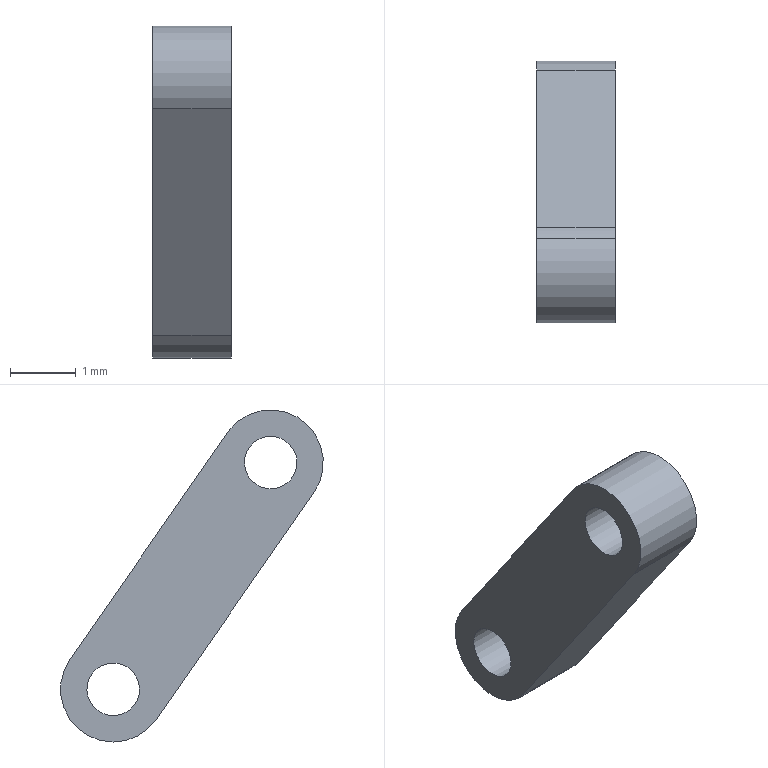Component | SolidWorks | FrontWingYoke-4 | 1 solid | 11 faces | box 1.2 x 4 x 5.05 mm | volume 9 mm3 | cylinder 7 | plane 4 | commonest cylinder face diameters 0.8 x4 1.6 x3
build123d program:
from build123d import *

# Parameters (mm, degrees)
SKETCH1_R           = 0.4
SKETCH1_R_2         = 0.4
BOSS_EXTRUDE1_DEPTH = 1.2


with BuildPart() as part:
    # Sketch1 → Boss-Extrude1 (new body)
    with BuildSketch(Plane.XY):
        with BuildLine():
            Line((7.129, 2.403), (8.391, 6.409))
            ThreePointArc((8.391, 6.409), (9.395, 6.931), (9.917, 5.928))
            Line((9.917, 5.928), (8.655, 1.922))
            ThreePointArc((8.655, 1.922), (7.652, 1.399), (7.129, 2.403))
        make_face()
        with Locations((7.892, 2.162)):
            Circle(SKETCH1_R, mode=Mode.SUBTRACT)
        with Locations((9.154, 6.168)):
            Circle(SKETCH1_R_2, mode=Mode.SUBTRACT)
    extrude(amount=BOSS_EXTRUDE1_DEPTH)


solid = part.part

# Placed as in the assembly
solid = solid.moved(Location((-5.1, 9.12, 5.065), (-37.732, 90, 0)))
STEP:
#1=CARTESIAN_POINT('',(-0.1535,0.2459,-0.08597));
#2=VERTEX_POINT('',#1);
#3=CARTESIAN_POINT('',(-0.1535,0.2266,-0.1109));
#4=VERTEX_POINT('',#3);
#5=CARTESIAN_POINT('',(-0.1535,0.2362,-0.09843));
#6=DIRECTION('',(1.,-0.,0.));
#7=DIRECTION('',(0.,-0.612,-0.7909));
#8=AXIS2_PLACEMENT_3D('',#5,#6,#7);
#9=CIRCLE('',#8,0.01575);
#10=EDGE_CURVE('',#2,#4,#9,.T.);
#11=ORIENTED_EDGE('',*,*,#10,.T.);
#12=CARTESIAN_POINT('',(-0.2008,0.2266,-0.1109));
#13=VERTEX_POINT('',#12);
#14=CARTESIAN_POINT('',(0.09426,0.2266,-0.1109));
#15=DIRECTION('',(-1.,0.,-0.));
#16=VECTOR('',#15,39.37);
#17=LINE('',#14,#16);
#18=EDGE_CURVE('',#4,#13,#17,.T.);
#19=ORIENTED_EDGE('',*,*,#18,.T.);
#20=CARTESIAN_POINT('',(-0.2008,0.2459,-0.08597));
#21=VERTEX_POINT('',#20);
#22=CARTESIAN_POINT('',(-0.2008,0.2362,-0.09843));
#23=DIRECTION('',(1.,-0.,0.));
#24=DIRECTION('',(0.,-0.612,-0.7909));
#25=AXIS2_PLACEMENT_3D('',#22,#23,#24);
#26=CIRCLE('',#25,0.01575);
#27=EDGE_CURVE('',#21,#13,#26,.T.);
#28=ORIENTED_EDGE('',*,*,#27,.F.);
#29=CARTESIAN_POINT('',(0.09426,0.2459,-0.08597));
#30=DIRECTION('',(-1.,0.,-0.));
#31=VECTOR('',#30,39.37);
#32=LINE('',#29,#31);
#33=EDGE_CURVE('',#2,#21,#32,.T.);
#34=ORIENTED_EDGE('',*,*,#33,.F.);
#35=EDGE_LOOP('',(#11,#19,#28,#34));
#36=FACE_OUTER_BOUND('',#35,.T.);
#37=CARTESIAN_POINT('',(0.09426,0.2362,-0.09843));
#38=DIRECTION('',(-1.,0.,-0.));
#39=DIRECTION('',(0.,0.612,0.7909));
#40=AXIS2_PLACEMENT_3D('',#37,#38,#39);
#41=CYLINDRICAL_SURFACE('',#40,0.01575);
#42=ADVANCED_FACE('',(#36),#41,.F.);
#43=CARTESIAN_POINT('',(-0.1535,0.2555,-0.07352));
#44=VERTEX_POINT('',#43);
#45=CARTESIAN_POINT('',(-0.1535,0.2104,-0.1164));
#46=VERTEX_POINT('',#45);
#47=CARTESIAN_POINT('',(-0.1535,0.2362,-0.09843));
#48=DIRECTION('',(1.,-0.,0.));
#49=DIRECTION('',(0.,-0.612,-0.7909));
#50=AXIS2_PLACEMENT_3D('',#47,#48,#49);
#51=CIRCLE('',#50,0.0315);
#52=EDGE_CURVE('',#44,#46,#51,.T.);
#53=ORIENTED_EDGE('',*,*,#52,.F.);
#54=CARTESIAN_POINT('',(-0.2008,0.2555,-0.07352));
#55=VERTEX_POINT('',#54);
#56=CARTESIAN_POINT('',(0.09426,0.2555,-0.07352));
#57=DIRECTION('',(-1.,0.,-0.));
#58=VECTOR('',#57,39.37);
#59=LINE('',#56,#58);
#60=EDGE_CURVE('',#44,#55,#59,.T.);
#61=ORIENTED_EDGE('',*,*,#60,.T.);
#62=CARTESIAN_POINT('',(-0.2008,0.2104,-0.1164));
#63=VERTEX_POINT('',#62);
#64=CARTESIAN_POINT('',(-0.2008,0.2362,-0.09843));
#65=DIRECTION('',(1.,-0.,0.));
#66=DIRECTION('',(0.,-0.612,-0.7909));
#67=AXIS2_PLACEMENT_3D('',#64,#65,#66);
#68=CIRCLE('',#67,0.0315);
#69=EDGE_CURVE('',#55,#63,#68,.T.);
#70=ORIENTED_EDGE('',*,*,#69,.T.);
#71=CARTESIAN_POINT('',(0.09426,0.2104,-0.1164));
#72=DIRECTION('',(-1.,0.,-0.));
#73=VECTOR('',#72,39.37);
#74=LINE('',#71,#73);
#75=EDGE_CURVE('',#46,#63,#74,.T.);
#76=ORIENTED_EDGE('',*,*,#75,.F.);
#77=EDGE_LOOP('',(#53,#61,#70,#76));
#78=FACE_OUTER_BOUND('',#77,.T.);
#79=CARTESIAN_POINT('',(0.09426,0.2362,-0.09843));
#80=DIRECTION('',(-1.,0.,-0.));
#81=DIRECTION('',(0.,0.612,0.7909));
#82=AXIS2_PLACEMENT_3D('',#79,#80,#81);
#83=CYLINDRICAL_SURFACE('',#82,0.0315);
#84=ADVANCED_FACE('',(#78),#83,.T.);
#85=CARTESIAN_POINT('',(-0.1535,0.3402,-0.2218));
#86=VERTEX_POINT('',#85);
#87=CARTESIAN_POINT('',(-0.1535,0.3209,-0.2467));
#88=VERTEX_POINT('',#87);
#89=CARTESIAN_POINT('',(-0.1535,0.3305,-0.2342));
#90=DIRECTION('',(1.,-0.,0.));
#91=DIRECTION('',(0.,-0.612,-0.7909));
#92=AXIS2_PLACEMENT_3D('',#89,#90,#91);
#93=CIRCLE('',#92,0.01575);
#94=EDGE_CURVE('',#86,#88,#93,.T.);
#95=ORIENTED_EDGE('',*,*,#94,.T.);
#96=CARTESIAN_POINT('',(-0.2008,0.3209,-0.2467));
#97=VERTEX_POINT('',#96);
#98=CARTESIAN_POINT('',(0.09426,0.3209,-0.2467));
#99=DIRECTION('',(-1.,0.,-0.));
#100=VECTOR('',#99,39.37);
#101=LINE('',#98,#100);
#102=EDGE_CURVE('',#88,#97,#101,.T.);
#103=ORIENTED_EDGE('',*,*,#102,.T.);
#104=CARTESIAN_POINT('',(-0.2008,0.3402,-0.2218));
#105=VERTEX_POINT('',#104);
#106=CARTESIAN_POINT('',(-0.2008,0.3305,-0.2342));
#107=DIRECTION('',(1.,-0.,0.));
#108=DIRECTION('',(0.,-0.612,-0.7909));
#109=AXIS2_PLACEMENT_3D('',#106,#107,#108);
#110=CIRCLE('',#109,0.01575);
#111=EDGE_CURVE('',#105,#97,#110,.T.);
#112=ORIENTED_EDGE('',*,*,#111,.F.);
#113=CARTESIAN_POINT('',(0.09426,0.3402,-0.2218));
#114=DIRECTION('',(-1.,0.,-0.));
#115=VECTOR('',#114,39.37);
#116=LINE('',#113,#115);
#117=EDGE_CURVE('',#86,#105,#116,.T.);
#118=ORIENTED_EDGE('',*,*,#117,.F.);
#119=EDGE_LOOP('',(#95,#103,#112,#118));
#120=FACE_OUTER_BOUND('',#119,.T.);
#121=CARTESIAN_POINT('',(0.09426,0.3305,-0.2342));
#122=DIRECTION('',(-1.,0.,-0.));
#123=DIRECTION('',(0.,0.612,0.7909));
#124=AXIS2_PLACEMENT_3D('',#121,#122,#123);
#125=CYLINDRICAL_SURFACE('',#124,0.01575);
#126=ADVANCED_FACE('',(#120),#125,.F.);
#127=ORIENTED_EDGE('',*,*,#102,.F.);
#128=CARTESIAN_POINT('',(-0.1535,0.3305,-0.2342));
#129=DIRECTION('',(1.,-0.,0.));
#130=DIRECTION('',(0.,-0.612,-0.7909));
#131=AXIS2_PLACEMENT_3D('',#128,#129,#130);
#132=CIRCLE('',#131,0.01575);
#133=EDGE_CURVE('',#88,#86,#132,.T.);
#134=ORIENTED_EDGE('',*,*,#133,.T.);
#135=ORIENTED_EDGE('',*,*,#117,.T.);
#136=CARTESIAN_POINT('',(-0.2008,0.3305,-0.2342));
#137=DIRECTION('',(1.,-0.,0.));
#138=DIRECTION('',(0.,-0.612,-0.7909));
#139=AXIS2_PLACEMENT_3D('',#136,#137,#138);
#140=CIRCLE('',#139,0.01575);
#141=EDGE_CURVE('',#97,#105,#140,.T.);
#142=ORIENTED_EDGE('',*,*,#141,.F.);
#143=EDGE_LOOP('',(#127,#134,#135,#142));
#144=FACE_OUTER_BOUND('',#143,.T.);
#145=CARTESIAN_POINT('',(0.09426,0.3305,-0.2342));
#146=DIRECTION('',(-1.,0.,-0.));
#147=DIRECTION('',(0.,0.612,0.7909));
#148=AXIS2_PLACEMENT_3D('',#145,#146,#147);
#149=CYLINDRICAL_SURFACE('',#148,0.01575);
#150=ADVANCED_FACE('',(#144),#149,.F.);
#151=CARTESIAN_POINT('',(-0.1535,0.3564,-0.2163));
#152=VERTEX_POINT('',#151);
#153=CARTESIAN_POINT('',(-0.1535,0.2621,-0.08046));
#154=VERTEX_POINT('',#153);
#155=CARTESIAN_POINT('',(-0.1535,0.2621,-0.08046));
#156=DIRECTION('',(-0.,-0.5704,0.8214));
#157=VECTOR('',#156,39.37);
#158=LINE('',#155,#157);
#159=EDGE_CURVE('',#152,#154,#158,.T.);
#160=ORIENTED_EDGE('',*,*,#159,.F.);
#161=CARTESIAN_POINT('',(-0.2008,0.3564,-0.2163));
#162=VERTEX_POINT('',#161);
#163=CARTESIAN_POINT('',(0.09426,0.3564,-0.2163));
#164=DIRECTION('',(-1.,0.,-0.));
#165=VECTOR('',#164,39.37);
#166=LINE('',#163,#165);
#167=EDGE_CURVE('',#152,#162,#166,.T.);
#168=ORIENTED_EDGE('',*,*,#167,.T.);
#169=CARTESIAN_POINT('',(-0.2008,0.2621,-0.08046));
#170=VERTEX_POINT('',#169);
#171=CARTESIAN_POINT('',(-0.2008,0.2621,-0.08046));
#172=DIRECTION('',(-0.,-0.5704,0.8214));
#173=VECTOR('',#172,39.37);
#174=LINE('',#171,#173);
#175=EDGE_CURVE('',#162,#170,#174,.T.);
#176=ORIENTED_EDGE('',*,*,#175,.T.);
#177=CARTESIAN_POINT('',(0.09426,0.2621,-0.08046));
#178=DIRECTION('',(-1.,0.,-0.));
#179=VECTOR('',#178,39.37);
#180=LINE('',#177,#179);
#181=EDGE_CURVE('',#154,#170,#180,.T.);
#182=ORIENTED_EDGE('',*,*,#181,.F.);
#183=EDGE_LOOP('',(#160,#168,#176,#182));
#184=FACE_OUTER_BOUND('',#183,.T.);
#185=CARTESIAN_POINT('',(0.09426,0.2621,-0.08046));
#186=DIRECTION('',(0.,-0.8214,-0.5704));
#187=DIRECTION('',(0.,0.5704,-0.8214));
#188=AXIS2_PLACEMENT_3D('',#185,#186,#187);
#189=PLANE('',#188);
#190=ADVANCED_FACE('',(#184),#189,.F.);
#191=CARTESIAN_POINT('',(-0.1535,0.3047,-0.2522));
#192=VERTEX_POINT('',#191);
#193=CARTESIAN_POINT('',(-0.1535,0.3305,-0.2342));
#194=DIRECTION('',(1.,-0.,0.));
#195=DIRECTION('',(0.,-0.612,-0.7909));
#196=AXIS2_PLACEMENT_3D('',#193,#194,#195);
#197=CIRCLE('',#196,0.0315);
#198=EDGE_CURVE('',#192,#152,#197,.T.);
#199=ORIENTED_EDGE('',*,*,#198,.F.);
#200=CARTESIAN_POINT('',(-0.2008,0.3047,-0.2522));
#201=VERTEX_POINT('',#200);
#202=CARTESIAN_POINT('',(0.09426,0.3047,-0.2522));
#203=DIRECTION('',(-1.,0.,-0.));
#204=VECTOR('',#203,39.37);
#205=LINE('',#202,#204);
#206=EDGE_CURVE('',#192,#201,#205,.T.);
#207=ORIENTED_EDGE('',*,*,#206,.T.);
#208=CARTESIAN_POINT('',(-0.2008,0.3305,-0.2342));
#209=DIRECTION('',(1.,-0.,0.));
#210=DIRECTION('',(0.,-0.612,-0.7909));
#211=AXIS2_PLACEMENT_3D('',#208,#209,#210);
#212=CIRCLE('',#211,0.0315);
#213=EDGE_CURVE('',#201,#162,#212,.T.);
#214=ORIENTED_EDGE('',*,*,#213,.T.);
#215=ORIENTED_EDGE('',*,*,#167,.F.);
#216=EDGE_LOOP('',(#199,#207,#214,#215));
#217=FACE_OUTER_BOUND('',#216,.T.);
#218=CARTESIAN_POINT('',(0.09426,0.3305,-0.2342));
#219=DIRECTION('',(-1.,0.,-0.));
#220=DIRECTION('',(0.,0.612,0.7909));
#221=AXIS2_PLACEMENT_3D('',#218,#219,#220);
#222=CYLINDRICAL_SURFACE('',#221,0.0315);
#223=ADVANCED_FACE('',(#217),#222,.T.);
#224=CARTESIAN_POINT('',(-0.1535,0.2104,-0.1164));
#225=DIRECTION('',(0.,0.5704,-0.8214));
#226=VECTOR('',#225,39.37);
#227=LINE('',#224,#226);
#228=EDGE_CURVE('',#46,#192,#227,.T.);
#229=ORIENTED_EDGE('',*,*,#228,.F.);
#230=ORIENTED_EDGE('',*,*,#75,.T.);
#231=CARTESIAN_POINT('',(-0.2008,0.2104,-0.1164));
#232=DIRECTION('',(0.,0.5704,-0.8214));
#233=VECTOR('',#232,39.37);
#234=LINE('',#231,#233);
#235=EDGE_CURVE('',#63,#201,#234,.T.);
#236=ORIENTED_EDGE('',*,*,#235,.T.);
#237=ORIENTED_EDGE('',*,*,#206,.F.);
#238=EDGE_LOOP('',(#229,#230,#236,#237));
#239=FACE_OUTER_BOUND('',#238,.T.);
#240=CARTESIAN_POINT('',(0.09426,0.2104,-0.1164));
#241=DIRECTION('',(-0.,0.8214,0.5704));
#242=DIRECTION('',(-0.,-0.5704,0.8214));
#243=AXIS2_PLACEMENT_3D('',#240,#241,#242);
#244=PLANE('',#243);
#245=ADVANCED_FACE('',(#239),#244,.F.);
#246=ORIENTED_EDGE('',*,*,#60,.F.);
#247=CARTESIAN_POINT('',(-0.1535,0.2362,-0.09843));
#248=DIRECTION('',(1.,-0.,0.));
#249=DIRECTION('',(0.,-0.612,-0.7909));
#250=AXIS2_PLACEMENT_3D('',#247,#248,#249);
#251=CIRCLE('',#250,0.0315);
#252=EDGE_CURVE('',#154,#44,#251,.T.);
#253=ORIENTED_EDGE('',*,*,#252,.F.);
#254=ORIENTED_EDGE('',*,*,#181,.T.);
#255=CARTESIAN_POINT('',(-0.2008,0.2362,-0.09843));
#256=DIRECTION('',(1.,-0.,0.));
#257=DIRECTION('',(0.,-0.612,-0.7909));
#258=AXIS2_PLACEMENT_3D('',#255,#256,#257);
#259=CIRCLE('',#258,0.0315);
#260=EDGE_CURVE('',#170,#55,#259,.T.);
#261=ORIENTED_EDGE('',*,*,#260,.T.);
#262=EDGE_LOOP('',(#246,#253,#254,#261));
#263=FACE_OUTER_BOUND('',#262,.T.);
#264=CARTESIAN_POINT('',(0.09426,0.2362,-0.09843));
#265=DIRECTION('',(-1.,0.,-0.));
#266=DIRECTION('',(0.,0.612,0.7909));
#267=AXIS2_PLACEMENT_3D('',#264,#265,#266);
#268=CYLINDRICAL_SURFACE('',#267,0.0315);
#269=ADVANCED_FACE('',(#263),#268,.T.);
#270=ORIENTED_EDGE('',*,*,#260,.F.);
#271=ORIENTED_EDGE('',*,*,#175,.F.);
#272=ORIENTED_EDGE('',*,*,#213,.F.);
#273=ORIENTED_EDGE('',*,*,#235,.F.);
#274=ORIENTED_EDGE('',*,*,#69,.F.);
#275=EDGE_LOOP('',(#270,#271,#272,#273,#274));
#276=FACE_OUTER_BOUND('',#275,.T.);
#277=ORIENTED_EDGE('',*,*,#111,.T.);
#278=ORIENTED_EDGE('',*,*,#141,.T.);
#279=EDGE_LOOP('',(#277,#278));
#280=FACE_BOUND('',#279,.T.);
#281=ORIENTED_EDGE('',*,*,#27,.T.);
#282=CARTESIAN_POINT('',(-0.2008,0.2362,-0.09843));
#283=DIRECTION('',(1.,-0.,0.));
#284=DIRECTION('',(0.,-0.612,-0.7909));
#285=AXIS2_PLACEMENT_3D('',#282,#283,#284);
#286=CIRCLE('',#285,0.01575);
#287=EDGE_CURVE('',#13,#21,#286,.T.);
#288=ORIENTED_EDGE('',*,*,#287,.T.);
#289=EDGE_LOOP('',(#281,#288));
#290=FACE_BOUND('',#289,.T.);
#291=CARTESIAN_POINT('',(-0.2008,0.2362,-0.09843));
#292=DIRECTION('',(1.,-0.,0.));
#293=DIRECTION('',(0.,-0.612,-0.7909));
#294=AXIS2_PLACEMENT_3D('',#291,#292,#293);
#295=PLANE('',#294);
#296=ADVANCED_FACE('',(#276,#280,#290),#295,.F.);
#297=ORIENTED_EDGE('',*,*,#18,.F.);
#298=CARTESIAN_POINT('',(-0.1535,0.2362,-0.09843));
#299=DIRECTION('',(1.,-0.,0.));
#300=DIRECTION('',(0.,-0.612,-0.7909));
#301=AXIS2_PLACEMENT_3D('',#298,#299,#300);
#302=CIRCLE('',#301,0.01575);
#303=EDGE_CURVE('',#4,#2,#302,.T.);
#304=ORIENTED_EDGE('',*,*,#303,.T.);
#305=ORIENTED_EDGE('',*,*,#33,.T.);
#306=ORIENTED_EDGE('',*,*,#287,.F.);
#307=EDGE_LOOP('',(#297,#304,#305,#306));
#308=FACE_OUTER_BOUND('',#307,.T.);
#309=CARTESIAN_POINT('',(0.09426,0.2362,-0.09843));
#310=DIRECTION('',(-1.,0.,-0.));
#311=DIRECTION('',(0.,0.612,0.7909));
#312=AXIS2_PLACEMENT_3D('',#309,#310,#311);
#313=CYLINDRICAL_SURFACE('',#312,0.01575);
#314=ADVANCED_FACE('',(#308),#313,.F.);
#315=ORIENTED_EDGE('',*,*,#10,.F.);
#316=ORIENTED_EDGE('',*,*,#303,.F.);
#317=EDGE_LOOP('',(#315,#316));
#318=FACE_BOUND('',#317,.T.);
#319=ORIENTED_EDGE('',*,*,#94,.F.);
#320=ORIENTED_EDGE('',*,*,#133,.F.);
#321=EDGE_LOOP('',(#319,#320));
#322=FACE_BOUND('',#321,.T.);
#323=ORIENTED_EDGE('',*,*,#159,.T.);
#324=ORIENTED_EDGE('',*,*,#252,.T.);
#325=ORIENTED_EDGE('',*,*,#52,.T.);
#326=ORIENTED_EDGE('',*,*,#228,.T.);
#327=ORIENTED_EDGE('',*,*,#198,.T.);
#328=EDGE_LOOP('',(#323,#324,#325,#326,#327));
#329=FACE_OUTER_BOUND('',#328,.T.);
#330=CARTESIAN_POINT('',(-0.1535,0.2931,-0.2075));
#331=DIRECTION('',(1.,-0.,0.));
#332=DIRECTION('',(0.,-0.612,-0.7909));
#333=AXIS2_PLACEMENT_3D('',#330,#331,#332);
#334=PLANE('',#333);
#335=ADVANCED_FACE('',(#318,#322,#329),#334,.T.);
#336=CLOSED_SHELL('',(#42,#84,#126,#150,#190,#223,#245,#269,#296,#314,#335));
#337=MANIFOLD_SOLID_BREP('',#336);
#338=CARTESIAN_POINT('',(0.,0.,0.));
#339=DIRECTION('',(0.,0.,1.));
#340=DIRECTION('',(1.,0.,0.));
#341=AXIS2_PLACEMENT_3D('',#338,#339,#340);
#342=(LENGTH_UNIT()NAMED_UNIT(*)SI_UNIT($,.METRE.));
#343=LENGTH_MEASURE_WITH_UNIT(LENGTH_MEASURE(0.0254),#342);
#344=DIMENSIONAL_EXPONENTS(1.,0.,0.,0.,0.,0.,0.);
#345=(CONVERSION_BASED_UNIT('',#343)LENGTH_UNIT()NAMED_UNIT(#344));
#346=UNCERTAINTY_MEASURE_WITH_UNIT(LENGTH_MEASURE(0.00001),#345,'','');
#347=(NAMED_UNIT(*)PLANE_ANGLE_UNIT()SI_UNIT($,.RADIAN.));
#348=(NAMED_UNIT(*)SI_UNIT($,.STERADIAN.)SOLID_ANGLE_UNIT());
#349=(GEOMETRIC_REPRESENTATION_CONTEXT(3)GLOBAL_UNCERTAINTY_ASSIGNED_CONTEXT((#346))GLOBAL_UNIT_ASSIGNED_CONTEXT((#345,#347,#348))REPRESENTATION_CONTEXT('',''));
#350=ADVANCED_BREP_SHAPE_REPRESENTATION('',(#337,#341),#349);
#351=COLOUR_RGB('',0.7922,0.8196,0.9333);
#352=FILL_AREA_STYLE_COLOUR('',#351);
#353=FILL_AREA_STYLE('',(#352));
#354=SURFACE_STYLE_FILL_AREA(#353);
#355=SURFACE_SIDE_STYLE('',(#354));
#356=SURFACE_STYLE_USAGE(.BOTH.,#355);
#357=PRESENTATION_STYLE_ASSIGNMENT((#356));
#358=STYLED_ITEM('',(#357),#337);
#359=(LENGTH_UNIT()NAMED_UNIT(*)SI_UNIT($,.METRE.));
#360=LENGTH_MEASURE_WITH_UNIT(LENGTH_MEASURE(0.0254),#359);
#361=DIMENSIONAL_EXPONENTS(1.,0.,0.,0.,0.,0.,0.);
#362=(CONVERSION_BASED_UNIT('',#360)LENGTH_UNIT()NAMED_UNIT(#361));
#363=UNCERTAINTY_MEASURE_WITH_UNIT(LENGTH_MEASURE(0.00001),#362,'','');
#364=(NAMED_UNIT(*)PLANE_ANGLE_UNIT()SI_UNIT($,.RADIAN.));
#365=(NAMED_UNIT(*)SI_UNIT($,.STERADIAN.)SOLID_ANGLE_UNIT());
#366=(GEOMETRIC_REPRESENTATION_CONTEXT(3)GLOBAL_UNCERTAINTY_ASSIGNED_CONTEXT((#363))GLOBAL_UNIT_ASSIGNED_CONTEXT((#362,#364,#365))REPRESENTATION_CONTEXT('',''));
#367=MECHANICAL_DESIGN_GEOMETRIC_PRESENTATION_REPRESENTATION('',(#358),#366);
#368=PRESENTATION_LAYER_ASSIGNMENT('','',(#358));